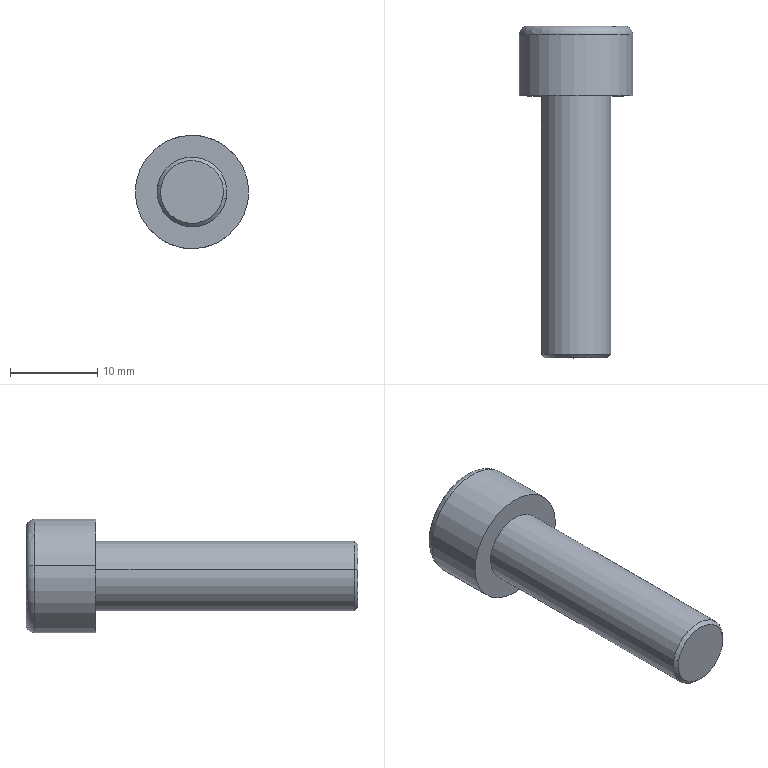Component | SolidWorks | hexagon socket head cap screws gb-25 | 1 solid | 25 faces | box 13 x 38 x 13 mm | volume 2418 mm3 | plane 15 | cone 4 | cylinder 4 | torus 2 | commonest cylinder face diameters 8 x2 13 x2
STEP:
#1=CARTESIAN_POINT('',(-5.304,20.394,23.936));
#2=VERTEX_POINT('',#1);
#3=CARTESIAN_POINT('',(-5.026,20.394,23.884));
#4=VERTEX_POINT('',#3);
#5=CARTESIAN_POINT('',(-5.165,20.394,23.91));
#6=DIRECTION('',(0.,-1.,0.));
#7=DIRECTION('',(-0.9828,0.,0.1847));
#8=AXIS2_PLACEMENT_3D('',#5,#6,#7);
#9=CIRCLE('',#8,0.1417);
#10=EDGE_CURVE('',#2,#4,#9,.T.);
#11=ORIENTED_EDGE('',*,*,#10,.F.);
#12=CARTESIAN_POINT('',(-5.32,20.41,23.939));
#13=VERTEX_POINT('',#12);
#14=CARTESIAN_POINT('',(-5.304,20.394,23.936));
#15=DIRECTION('',(-0.6949,0.7071,0.1306));
#16=VECTOR('',#15,39.37);
#17=LINE('',#14,#16);
#18=EDGE_CURVE('',#2,#13,#17,.T.);
#19=ORIENTED_EDGE('',*,*,#18,.T.);
#20=CARTESIAN_POINT('',(-5.01,20.41,23.881));
#21=VERTEX_POINT('',#20);
#22=CARTESIAN_POINT('',(-5.165,20.41,23.91));
#23=DIRECTION('',(0.,1.,0.));
#24=DIRECTION('',(-0.9828,0.,0.1847));
#25=AXIS2_PLACEMENT_3D('',#22,#23,#24);
#26=CIRCLE('',#25,0.1575);
#27=EDGE_CURVE('',#21,#13,#26,.T.);
#28=ORIENTED_EDGE('',*,*,#27,.F.);
#29=CARTESIAN_POINT('',(-5.026,20.394,23.884));
#30=DIRECTION('',(0.6949,0.7071,-0.1306));
#31=VECTOR('',#30,39.37);
#32=LINE('',#29,#31);
#33=EDGE_CURVE('',#4,#21,#32,.T.);
#34=ORIENTED_EDGE('',*,*,#33,.F.);
#35=EDGE_LOOP('',(#11,#19,#28,#34));
#36=FACE_OUTER_BOUND('',#35,.T.);
#37=CARTESIAN_POINT('',(-5.165,20.394,23.91));
#38=DIRECTION('',(0.,1.,0.));
#39=DIRECTION('',(0.9828,0.,-0.1847));
#40=AXIS2_PLACEMENT_3D('',#37,#38,#39);
#41=CONICAL_SURFACE('',#40,0.1417,0.7854);
#42=ADVANCED_FACE('',(#36),#41,.T.);
#43=CARTESIAN_POINT('',(-4.952,21.891,23.87));
#44=VERTEX_POINT('',#43);
#45=CARTESIAN_POINT('',(-5.378,21.891,23.95));
#46=VERTEX_POINT('',#45);
#47=CARTESIAN_POINT('',(-5.165,21.891,23.91));
#48=DIRECTION('',(0.,1.,0.));
#49=DIRECTION('',(-0.9828,0.,0.1847));
#50=AXIS2_PLACEMENT_3D('',#47,#48,#49);
#51=CIRCLE('',#50,0.2165);
#52=EDGE_CURVE('',#44,#46,#51,.T.);
#53=ORIENTED_EDGE('',*,*,#52,.F.);
#54=CARTESIAN_POINT('',(-4.913,21.851,23.863));
#55=VERTEX_POINT('',#54);
#56=CARTESIAN_POINT('',(-4.952,21.851,23.87));
#57=DIRECTION('',(-0.1847,0.,-0.9828));
#58=DIRECTION('',(-0.9828,0.,0.1847));
#59=AXIS2_PLACEMENT_3D('',#56,#57,#58);
#60=CIRCLE('',#59,0.03937);
#61=EDGE_CURVE('',#44,#55,#60,.T.);
#62=ORIENTED_EDGE('',*,*,#61,.T.);
#63=CARTESIAN_POINT('',(-5.416,21.851,23.957));
#64=VERTEX_POINT('',#63);
#65=CARTESIAN_POINT('',(-5.165,21.851,23.91));
#66=DIRECTION('',(0.,-1.,0.));
#67=DIRECTION('',(-0.9828,0.,0.1847));
#68=AXIS2_PLACEMENT_3D('',#65,#66,#67);
#69=CIRCLE('',#68,0.2559);
#70=EDGE_CURVE('',#64,#55,#69,.T.);
#71=ORIENTED_EDGE('',*,*,#70,.F.);
#72=CARTESIAN_POINT('',(-5.378,21.851,23.95));
#73=DIRECTION('',(0.1847,0.,0.9828));
#74=DIRECTION('',(0.9828,0.,-0.1847));
#75=AXIS2_PLACEMENT_3D('',#72,#73,#74);
#76=CIRCLE('',#75,0.03937);
#77=EDGE_CURVE('',#46,#64,#76,.T.);
#78=ORIENTED_EDGE('',*,*,#77,.F.);
#79=EDGE_LOOP('',(#53,#62,#71,#78));
#80=FACE_OUTER_BOUND('',#79,.T.);
#81=CARTESIAN_POINT('',(-5.165,21.851,23.91));
#82=DIRECTION('',(0.,-1.,0.));
#83=DIRECTION('',(-0.9828,0.,0.1847));
#84=AXIS2_PLACEMENT_3D('',#81,#82,#83);
#85=TOROIDAL_SURFACE('',#84,0.2165,0.03937);
#86=ADVANCED_FACE('',(#80),#85,.T.);
#87=CARTESIAN_POINT('',(-5.165,21.665,23.91));
#88=VERTEX_POINT('',#87);
#89=CARTESIAN_POINT('',(-5.049,21.733,23.888));
#90=VERTEX_POINT('',#89);
#91=CARTESIAN_POINT('',(-5.049,21.733,23.888));
#92=DIRECTION('',(0.8511,0.5,-0.16));
#93=VECTOR('',#92,39.37);
#94=LINE('',#91,#93);
#95=EDGE_CURVE('',#88,#90,#94,.T.);
#96=ORIENTED_EDGE('',*,*,#95,.F.);
#97=CARTESIAN_POINT('',(-5.281,21.733,23.932));
#98=VERTEX_POINT('',#97);
#99=CARTESIAN_POINT('',(-5.281,21.733,23.932));
#100=DIRECTION('',(-0.8511,0.5,0.16));
#101=VECTOR('',#100,39.37);
#102=LINE('',#99,#101);
#103=EDGE_CURVE('',#88,#98,#102,.T.);
#104=ORIENTED_EDGE('',*,*,#103,.T.);
#105=CARTESIAN_POINT('',(-5.255,21.733,23.987));
#106=VERTEX_POINT('',#105);
#107=CARTESIAN_POINT('',(-5.165,21.733,23.91));
#108=DIRECTION('',(0.,-1.,0.));
#109=DIRECTION('',(0.9828,0.,-0.1847));
#110=AXIS2_PLACEMENT_3D('',#107,#108,#109);
#111=CIRCLE('',#110,0.1181);
#112=EDGE_CURVE('',#106,#98,#111,.T.);
#113=ORIENTED_EDGE('',*,*,#112,.F.);
#114=CARTESIAN_POINT('',(-5.143,21.733,24.026));
#115=VERTEX_POINT('',#114);
#116=CARTESIAN_POINT('',(-5.165,21.733,23.91));
#117=DIRECTION('',(0.,-1.,0.));
#118=DIRECTION('',(0.9828,0.,-0.1847));
#119=AXIS2_PLACEMENT_3D('',#116,#117,#118);
#120=CIRCLE('',#119,0.1181);
#121=EDGE_CURVE('',#115,#106,#120,.T.);
#122=ORIENTED_EDGE('',*,*,#121,.F.);
#123=CARTESIAN_POINT('',(-5.054,21.733,23.949));
#124=VERTEX_POINT('',#123);
#125=CARTESIAN_POINT('',(-5.165,21.733,23.91));
#126=DIRECTION('',(0.,-1.,0.));
#127=DIRECTION('',(0.9828,0.,-0.1847));
#128=AXIS2_PLACEMENT_3D('',#125,#126,#127);
#129=CIRCLE('',#128,0.1181);
#130=EDGE_CURVE('',#124,#115,#129,.T.);
#131=ORIENTED_EDGE('',*,*,#130,.F.);
#132=CARTESIAN_POINT('',(-5.165,21.733,23.91));
#133=DIRECTION('',(0.,-1.,0.));
#134=DIRECTION('',(0.9828,0.,-0.1847));
#135=AXIS2_PLACEMENT_3D('',#132,#133,#134);
#136=CIRCLE('',#135,0.1181);
#137=EDGE_CURVE('',#90,#124,#136,.T.);
#138=ORIENTED_EDGE('',*,*,#137,.F.);
#139=EDGE_LOOP('',(#96,#104,#113,#122,#131,#138));
#140=FACE_OUTER_BOUND('',#139,.T.);
#141=CARTESIAN_POINT('',(-5.165,21.733,23.91));
#142=DIRECTION('',(0.,1.,0.));
#143=DIRECTION('',(0.9828,0.,-0.1847));
#144=AXIS2_PLACEMENT_3D('',#141,#142,#143);
#145=CONICAL_SURFACE('',#144,0.1181,1.047);
#146=ADVANCED_FACE('',(#140),#145,.F.);
#147=ORIENTED_EDGE('',*,*,#27,.T.);
#148=CARTESIAN_POINT('',(-5.32,21.576,23.939));
#149=VERTEX_POINT('',#148);
#150=CARTESIAN_POINT('',(-5.32,20.394,23.939));
#151=DIRECTION('',(0.,1.,0.));
#152=VECTOR('',#151,39.37);
#153=LINE('',#150,#152);
#154=EDGE_CURVE('',#13,#149,#153,.T.);
#155=ORIENTED_EDGE('',*,*,#154,.T.);
#156=CARTESIAN_POINT('',(-5.01,21.576,23.881));
#157=VERTEX_POINT('',#156);
#158=CARTESIAN_POINT('',(-5.165,21.576,23.91));
#159=DIRECTION('',(0.,-1.,0.));
#160=DIRECTION('',(-0.9828,0.,0.1847));
#161=AXIS2_PLACEMENT_3D('',#158,#159,#160);
#162=CIRCLE('',#161,0.1575);
#163=EDGE_CURVE('',#149,#157,#162,.T.);
#164=ORIENTED_EDGE('',*,*,#163,.T.);
#165=CARTESIAN_POINT('',(-5.01,20.394,23.881));
#166=DIRECTION('',(0.,1.,0.));
#167=VECTOR('',#166,39.37);
#168=LINE('',#165,#167);
#169=EDGE_CURVE('',#21,#157,#168,.T.);
#170=ORIENTED_EDGE('',*,*,#169,.F.);
#171=EDGE_LOOP('',(#147,#155,#164,#170));
#172=FACE_OUTER_BOUND('',#171,.T.);
#173=CARTESIAN_POINT('',(-5.165,20.394,23.91));
#174=DIRECTION('',(0.,1.,0.));
#175=DIRECTION('',(0.9828,0.,-0.1847));
#176=AXIS2_PLACEMENT_3D('',#173,#174,#175);
#177=CYLINDRICAL_SURFACE('',#176,0.1575);
#178=ADVANCED_FACE('',(#172),#177,.T.);
#179=CARTESIAN_POINT('',(-5.416,21.576,23.957));
#180=VERTEX_POINT('',#179);
#181=CARTESIAN_POINT('',(-4.913,21.576,23.863));
#182=VERTEX_POINT('',#181);
#183=CARTESIAN_POINT('',(-5.165,21.576,23.91));
#184=DIRECTION('',(0.,-1.,0.));
#185=DIRECTION('',(-0.9828,0.,0.1847));
#186=AXIS2_PLACEMENT_3D('',#183,#184,#185);
#187=CIRCLE('',#186,0.2559);
#188=EDGE_CURVE('',#180,#182,#187,.T.);
#189=ORIENTED_EDGE('',*,*,#188,.F.);
#190=CARTESIAN_POINT('',(-5.416,21.576,23.957));
#191=DIRECTION('',(0.,1.,0.));
#192=VECTOR('',#191,39.37);
#193=LINE('',#190,#192);
#194=EDGE_CURVE('',#180,#64,#193,.T.);
#195=ORIENTED_EDGE('',*,*,#194,.T.);
#196=ORIENTED_EDGE('',*,*,#70,.T.);
#197=CARTESIAN_POINT('',(-4.913,21.576,23.863));
#198=DIRECTION('',(0.,1.,0.));
#199=VECTOR('',#198,39.37);
#200=LINE('',#197,#199);
#201=EDGE_CURVE('',#182,#55,#200,.T.);
#202=ORIENTED_EDGE('',*,*,#201,.F.);
#203=EDGE_LOOP('',(#189,#195,#196,#202));
#204=FACE_OUTER_BOUND('',#203,.T.);
#205=CARTESIAN_POINT('',(-5.165,21.576,23.91));
#206=DIRECTION('',(0.,1.,0.));
#207=DIRECTION('',(0.9828,0.,-0.1847));
#208=AXIS2_PLACEMENT_3D('',#205,#206,#207);
#209=CYLINDRICAL_SURFACE('',#208,0.2559);
#210=ADVANCED_FACE('',(#204),#209,.T.);
#211=CARTESIAN_POINT('',(-5.076,21.733,24.013));
#212=VERTEX_POINT('',#211);
#213=CARTESIAN_POINT('',(-5.031,21.733,23.885));
#214=DIRECTION('',(-0.3314,0.,0.9435));
#215=VECTOR('',#214,39.37);
#216=LINE('',#213,#215);
#217=EDGE_CURVE('',#124,#212,#216,.T.);
#218=ORIENTED_EDGE('',*,*,#217,.F.);
#219=ORIENTED_EDGE('',*,*,#130,.T.);
#220=CARTESIAN_POINT('',(-5.076,21.733,24.013));
#221=DIRECTION('',(-0.9828,0.,0.1847));
#222=VECTOR('',#221,39.37);
#223=LINE('',#220,#222);
#224=EDGE_CURVE('',#212,#115,#223,.T.);
#225=ORIENTED_EDGE('',*,*,#224,.F.);
#226=EDGE_LOOP('',(#218,#219,#225));
#227=FACE_OUTER_BOUND('',#226,.T.);
#228=CARTESIAN_POINT('',(-5.121,21.733,24.142));
#229=DIRECTION('',(0.,1.,0.));
#230=DIRECTION('',(0.9828,0.,-0.1847));
#231=AXIS2_PLACEMENT_3D('',#228,#229,#230);
#232=PLANE('',#231);
#233=ADVANCED_FACE('',(#227),#232,.T.);
#234=CARTESIAN_POINT('',(-5.21,21.733,24.039));
#235=VERTEX_POINT('',#234);
#236=CARTESIAN_POINT('',(-5.076,21.733,24.013));
#237=DIRECTION('',(-0.9828,0.,0.1847));
#238=VECTOR('',#237,39.37);
#239=LINE('',#236,#238);
#240=EDGE_CURVE('',#115,#235,#239,.T.);
#241=ORIENTED_EDGE('',*,*,#240,.F.);
#242=ORIENTED_EDGE('',*,*,#121,.T.);
#243=CARTESIAN_POINT('',(-5.21,21.733,24.039));
#244=DIRECTION('',(-0.6513,0.,-0.7588));
#245=VECTOR('',#244,39.37);
#246=LINE('',#243,#245);
#247=EDGE_CURVE('',#235,#106,#246,.T.);
#248=ORIENTED_EDGE('',*,*,#247,.F.);
#249=EDGE_LOOP('',(#241,#242,#248));
#250=FACE_OUTER_BOUND('',#249,.T.);
#251=CARTESIAN_POINT('',(-5.121,21.733,24.142));
#252=DIRECTION('',(0.,1.,0.));
#253=DIRECTION('',(0.9828,0.,-0.1847));
#254=AXIS2_PLACEMENT_3D('',#251,#252,#253);
#255=PLANE('',#254);
#256=ADVANCED_FACE('',(#250),#255,.T.);
#257=CARTESIAN_POINT('',(-5.299,21.733,23.935));
#258=VERTEX_POINT('',#257);
#259=CARTESIAN_POINT('',(-5.21,21.733,24.039));
#260=DIRECTION('',(-0.6513,0.,-0.7588));
#261=VECTOR('',#260,39.37);
#262=LINE('',#259,#261);
#263=EDGE_CURVE('',#106,#258,#262,.T.);
#264=ORIENTED_EDGE('',*,*,#263,.F.);
#265=ORIENTED_EDGE('',*,*,#112,.T.);
#266=CARTESIAN_POINT('',(-5.276,21.733,23.871));
#267=VERTEX_POINT('',#266);
#268=CARTESIAN_POINT('',(-5.165,21.733,23.91));
#269=DIRECTION('',(0.,-1.,0.));
#270=DIRECTION('',(0.9828,0.,-0.1847));
#271=AXIS2_PLACEMENT_3D('',#268,#269,#270);
#272=CIRCLE('',#271,0.1181);
#273=EDGE_CURVE('',#98,#267,#272,.T.);
#274=ORIENTED_EDGE('',*,*,#273,.T.);
#275=CARTESIAN_POINT('',(-5.299,21.733,23.935));
#276=DIRECTION('',(0.3314,0.,-0.9435));
#277=VECTOR('',#276,39.37);
#278=LINE('',#275,#277);
#279=EDGE_CURVE('',#258,#267,#278,.T.);
#280=ORIENTED_EDGE('',*,*,#279,.F.);
#281=EDGE_LOOP('',(#264,#265,#274,#280));
#282=FACE_OUTER_BOUND('',#281,.T.);
#283=CARTESIAN_POINT('',(-5.121,21.733,24.142));
#284=DIRECTION('',(0.,1.,0.));
#285=DIRECTION('',(0.9828,0.,-0.1847));
#286=AXIS2_PLACEMENT_3D('',#283,#284,#285);
#287=PLANE('',#286);
#288=ADVANCED_FACE('',(#282),#287,.T.);
#289=CARTESIAN_POINT('',(-5.254,21.733,23.806));
#290=VERTEX_POINT('',#289);
#291=CARTESIAN_POINT('',(-5.299,21.733,23.935));
#292=DIRECTION('',(0.3314,0.,-0.9435));
#293=VECTOR('',#292,39.37);
#294=LINE('',#291,#293);
#295=EDGE_CURVE('',#267,#290,#294,.T.);
#296=ORIENTED_EDGE('',*,*,#295,.F.);
#297=CARTESIAN_POINT('',(-5.187,21.733,23.794));
#298=VERTEX_POINT('',#297);
#299=CARTESIAN_POINT('',(-5.165,21.733,23.91));
#300=DIRECTION('',(0.,-1.,0.));
#301=DIRECTION('',(-0.9828,0.,0.1847));
#302=AXIS2_PLACEMENT_3D('',#299,#300,#301);
#303=CIRCLE('',#302,0.1181);
#304=EDGE_CURVE('',#267,#298,#303,.T.);
#305=ORIENTED_EDGE('',*,*,#304,.T.);
#306=CARTESIAN_POINT('',(-5.254,21.733,23.806));
#307=DIRECTION('',(0.9828,0.,-0.1847));
#308=VECTOR('',#307,39.37);
#309=LINE('',#306,#308);
#310=EDGE_CURVE('',#290,#298,#309,.T.);
#311=ORIENTED_EDGE('',*,*,#310,.F.);
#312=EDGE_LOOP('',(#296,#305,#311));
#313=FACE_OUTER_BOUND('',#312,.T.);
#314=CARTESIAN_POINT('',(-5.121,21.733,24.142));
#315=DIRECTION('',(0.,1.,0.));
#316=DIRECTION('',(0.9828,0.,-0.1847));
#317=AXIS2_PLACEMENT_3D('',#314,#315,#316);
#318=PLANE('',#317);
#319=ADVANCED_FACE('',(#313),#318,.T.);
#320=CARTESIAN_POINT('',(-5.12,21.733,23.781));
#321=VERTEX_POINT('',#320);
#322=CARTESIAN_POINT('',(-5.254,21.733,23.806));
#323=DIRECTION('',(0.9828,0.,-0.1847));
#324=VECTOR('',#323,39.37);
#325=LINE('',#322,#324);
#326=EDGE_CURVE('',#298,#321,#325,.T.);
#327=ORIENTED_EDGE('',*,*,#326,.F.);
#328=CARTESIAN_POINT('',(-5.075,21.733,23.833));
#329=VERTEX_POINT('',#328);
#330=CARTESIAN_POINT('',(-5.165,21.733,23.91));
#331=DIRECTION('',(0.,-1.,0.));
#332=DIRECTION('',(0.9828,0.,-0.1847));
#333=AXIS2_PLACEMENT_3D('',#330,#331,#332);
#334=CIRCLE('',#333,0.1181);
#335=EDGE_CURVE('',#298,#329,#334,.T.);
#336=ORIENTED_EDGE('',*,*,#335,.T.);
#337=CARTESIAN_POINT('',(-5.12,21.733,23.781));
#338=DIRECTION('',(0.6513,0.,0.7588));
#339=VECTOR('',#338,39.37);
#340=LINE('',#337,#339);
#341=EDGE_CURVE('',#321,#329,#340,.T.);
#342=ORIENTED_EDGE('',*,*,#341,.F.);
#343=EDGE_LOOP('',(#327,#336,#342));
#344=FACE_OUTER_BOUND('',#343,.T.);
#345=CARTESIAN_POINT('',(-5.121,21.733,24.142));
#346=DIRECTION('',(0.,1.,0.));
#347=DIRECTION('',(0.9828,0.,-0.1847));
#348=AXIS2_PLACEMENT_3D('',#345,#346,#347);
#349=PLANE('',#348);
#350=ADVANCED_FACE('',(#344),#349,.T.);
#351=CARTESIAN_POINT('',(-5.031,21.733,23.885));
#352=VERTEX_POINT('',#351);
#353=CARTESIAN_POINT('',(-5.12,21.733,23.781));
#354=DIRECTION('',(0.6513,0.,0.7588));
#355=VECTOR('',#354,39.37);
#356=LINE('',#353,#355);
#357=EDGE_CURVE('',#329,#352,#356,.T.);
#358=ORIENTED_EDGE('',*,*,#357,.F.);
#359=CARTESIAN_POINT('',(-5.165,21.733,23.91));
#360=DIRECTION('',(0.,-1.,0.));
#361=DIRECTION('',(0.9828,0.,-0.1847));
#362=AXIS2_PLACEMENT_3D('',#359,#360,#361);
#363=CIRCLE('',#362,0.1181);
#364=EDGE_CURVE('',#329,#90,#363,.T.);
#365=ORIENTED_EDGE('',*,*,#364,.T.);
#366=ORIENTED_EDGE('',*,*,#137,.T.);
#367=CARTESIAN_POINT('',(-5.031,21.733,23.885));
#368=DIRECTION('',(-0.3314,0.,0.9435));
#369=VECTOR('',#368,39.37);
#370=LINE('',#367,#369);
#371=EDGE_CURVE('',#352,#124,#370,.T.);
#372=ORIENTED_EDGE('',*,*,#371,.F.);
#373=EDGE_LOOP('',(#358,#365,#366,#372));
#374=FACE_OUTER_BOUND('',#373,.T.);
#375=CARTESIAN_POINT('',(-5.121,21.733,24.142));
#376=DIRECTION('',(0.,1.,0.));
#377=DIRECTION('',(0.9828,0.,-0.1847));
#378=AXIS2_PLACEMENT_3D('',#375,#376,#377);
#379=PLANE('',#378);
#380=ADVANCED_FACE('',(#374),#379,.T.);
#381=CARTESIAN_POINT('',(-5.165,21.891,23.91));
#382=DIRECTION('',(0.,1.,0.));
#383=DIRECTION('',(-0.9828,0.,0.1847));
#384=AXIS2_PLACEMENT_3D('',#381,#382,#383);
#385=CIRCLE('',#384,0.2165);
#386=EDGE_CURVE('',#46,#44,#385,.T.);
#387=ORIENTED_EDGE('',*,*,#386,.T.);
#388=ORIENTED_EDGE('',*,*,#52,.T.);
#389=EDGE_LOOP('',(#387,#388));
#390=FACE_OUTER_BOUND('',#389,.T.);
#391=CARTESIAN_POINT('',(-5.21,21.891,24.039));
#392=VERTEX_POINT('',#391);
#393=CARTESIAN_POINT('',(-5.299,21.891,23.935));
#394=VERTEX_POINT('',#393);
#395=CARTESIAN_POINT('',(-5.21,21.891,24.039));
#396=DIRECTION('',(-0.6513,0.,-0.7588));
#397=VECTOR('',#396,39.37);
#398=LINE('',#395,#397);
#399=EDGE_CURVE('',#392,#394,#398,.T.);
#400=ORIENTED_EDGE('',*,*,#399,.T.);
#401=CARTESIAN_POINT('',(-5.254,21.891,23.806));
#402=VERTEX_POINT('',#401);
#403=CARTESIAN_POINT('',(-5.299,21.891,23.935));
#404=DIRECTION('',(0.3314,0.,-0.9435));
#405=VECTOR('',#404,39.37);
#406=LINE('',#403,#405);
#407=EDGE_CURVE('',#394,#402,#406,.T.);
#408=ORIENTED_EDGE('',*,*,#407,.T.);
#409=CARTESIAN_POINT('',(-5.12,21.891,23.781));
#410=VERTEX_POINT('',#409);
#411=CARTESIAN_POINT('',(-5.254,21.891,23.806));
#412=DIRECTION('',(0.9828,0.,-0.1847));
#413=VECTOR('',#412,39.37);
#414=LINE('',#411,#413);
#415=EDGE_CURVE('',#402,#410,#414,.T.);
#416=ORIENTED_EDGE('',*,*,#415,.T.);
#417=CARTESIAN_POINT('',(-5.031,21.891,23.885));
#418=VERTEX_POINT('',#417);
#419=CARTESIAN_POINT('',(-5.12,21.891,23.781));
#420=DIRECTION('',(0.6513,0.,0.7588));
#421=VECTOR('',#420,39.37);
#422=LINE('',#419,#421);
#423=EDGE_CURVE('',#410,#418,#422,.T.);
#424=ORIENTED_EDGE('',*,*,#423,.T.);
#425=CARTESIAN_POINT('',(-5.076,21.891,24.013));
#426=VERTEX_POINT('',#425);
#427=CARTESIAN_POINT('',(-5.031,21.891,23.885));
#428=DIRECTION('',(-0.3314,0.,0.9435));
#429=VECTOR('',#428,39.37);
#430=LINE('',#427,#429);
#431=EDGE_CURVE('',#418,#426,#430,.T.);
#432=ORIENTED_EDGE('',*,*,#431,.T.);
#433=CARTESIAN_POINT('',(-5.076,21.891,24.013));
#434=DIRECTION('',(-0.9828,0.,0.1847));
#435=VECTOR('',#434,39.37);
#436=LINE('',#433,#435);
#437=EDGE_CURVE('',#426,#392,#436,.T.);
#438=ORIENTED_EDGE('',*,*,#437,.T.);
#439=EDGE_LOOP('',(#400,#408,#416,#424,#432,#438));
#440=FACE_BOUND('',#439,.T.);
#441=CARTESIAN_POINT('',(-5.165,21.891,23.91));
#442=DIRECTION('',(0.,-1.,0.));
#443=DIRECTION('',(-0.9828,0.,0.1847));
#444=AXIS2_PLACEMENT_3D('',#441,#442,#443);
#445=PLANE('',#444);
#446=ADVANCED_FACE('',(#390,#440),#445,.F.);
#447=CARTESIAN_POINT('',(-5.165,21.576,23.91));
#448=DIRECTION('',(0.,-1.,0.));
#449=DIRECTION('',(-0.9828,0.,0.1847));
#450=AXIS2_PLACEMENT_3D('',#447,#448,#449);
#451=CIRCLE('',#450,0.2559);
#452=EDGE_CURVE('',#182,#180,#451,.T.);
#453=ORIENTED_EDGE('',*,*,#452,.T.);
#454=ORIENTED_EDGE('',*,*,#188,.T.);
#455=EDGE_LOOP('',(#453,#454));
#456=FACE_OUTER_BOUND('',#455,.T.);
#457=CARTESIAN_POINT('',(-5.165,21.576,23.91));
#458=DIRECTION('',(0.,-1.,0.));
#459=DIRECTION('',(-0.9828,0.,0.1847));
#460=AXIS2_PLACEMENT_3D('',#457,#458,#459);
#461=CIRCLE('',#460,0.1575);
#462=EDGE_CURVE('',#157,#149,#461,.T.);
#463=ORIENTED_EDGE('',*,*,#462,.F.);
#464=ORIENTED_EDGE('',*,*,#163,.F.);
#465=EDGE_LOOP('',(#463,#464));
#466=FACE_BOUND('',#465,.T.);
#467=CARTESIAN_POINT('',(-5.165,21.576,23.91));
#468=DIRECTION('',(0.,-1.,0.));
#469=DIRECTION('',(-0.9828,0.,0.1847));
#470=AXIS2_PLACEMENT_3D('',#467,#468,#469);
#471=PLANE('',#470);
#472=ADVANCED_FACE('',(#456,#466),#471,.T.);
#473=ORIENTED_EDGE('',*,*,#194,.F.);
#474=ORIENTED_EDGE('',*,*,#452,.F.);
#475=ORIENTED_EDGE('',*,*,#201,.T.);
#476=CARTESIAN_POINT('',(-5.165,21.851,23.91));
#477=DIRECTION('',(0.,-1.,0.));
#478=DIRECTION('',(-0.9828,0.,0.1847));
#479=AXIS2_PLACEMENT_3D('',#476,#477,#478);
#480=CIRCLE('',#479,0.2559);
#481=EDGE_CURVE('',#55,#64,#480,.T.);
#482=ORIENTED_EDGE('',*,*,#481,.T.);
#483=EDGE_LOOP('',(#473,#474,#475,#482));
#484=FACE_OUTER_BOUND('',#483,.T.);
#485=CARTESIAN_POINT('',(-5.165,21.576,23.91));
#486=DIRECTION('',(0.,1.,0.));
#487=DIRECTION('',(0.9828,0.,-0.1847));
#488=AXIS2_PLACEMENT_3D('',#485,#486,#487);
#489=CYLINDRICAL_SURFACE('',#488,0.2559);
#490=ADVANCED_FACE('',(#484),#489,.T.);
#491=ORIENTED_EDGE('',*,*,#154,.F.);
#492=CARTESIAN_POINT('',(-5.165,20.41,23.91));
#493=DIRECTION('',(0.,1.,0.));
#494=DIRECTION('',(-0.9828,0.,0.1847));
#495=AXIS2_PLACEMENT_3D('',#492,#493,#494);
#496=CIRCLE('',#495,0.1575);
#497=EDGE_CURVE('',#13,#21,#496,.T.);
#498=ORIENTED_EDGE('',*,*,#497,.T.);
#499=ORIENTED_EDGE('',*,*,#169,.T.);
#500=ORIENTED_EDGE('',*,*,#462,.T.);
#501=EDGE_LOOP('',(#491,#498,#499,#500));
#502=FACE_OUTER_BOUND('',#501,.T.);
#503=CARTESIAN_POINT('',(-5.165,20.394,23.91));
#504=DIRECTION('',(0.,1.,0.));
#505=DIRECTION('',(0.9828,0.,-0.1847));
#506=AXIS2_PLACEMENT_3D('',#503,#504,#505);
#507=CYLINDRICAL_SURFACE('',#506,0.1575);
#508=ADVANCED_FACE('',(#502),#507,.T.);
#509=CARTESIAN_POINT('',(-5.165,20.394,23.91));
#510=DIRECTION('',(0.,-1.,0.));
#511=DIRECTION('',(-0.9828,0.,0.1847));
#512=AXIS2_PLACEMENT_3D('',#509,#510,#511);
#513=CIRCLE('',#512,0.1417);
#514=EDGE_CURVE('',#4,#2,#513,.T.);
#515=ORIENTED_EDGE('',*,*,#514,.T.);
#516=ORIENTED_EDGE('',*,*,#10,.T.);
#517=EDGE_LOOP('',(#515,#516));
#518=FACE_OUTER_BOUND('',#517,.T.);
#519=CARTESIAN_POINT('',(-5.165,20.394,23.91));
#520=DIRECTION('',(0.,-1.,0.));
#521=DIRECTION('',(-0.9828,0.,0.1847));
#522=AXIS2_PLACEMENT_3D('',#519,#520,#521);
#523=PLANE('',#522);
#524=ADVANCED_FACE('',(#518),#523,.T.);
#525=ORIENTED_EDGE('',*,*,#399,.F.);
#526=CARTESIAN_POINT('',(-5.21,21.733,24.039));
#527=DIRECTION('',(0.,1.,0.));
#528=VECTOR('',#527,39.37);
#529=LINE('',#526,#528);
#530=EDGE_CURVE('',#235,#392,#529,.T.);
#531=ORIENTED_EDGE('',*,*,#530,.F.);
#532=ORIENTED_EDGE('',*,*,#247,.T.);
#533=ORIENTED_EDGE('',*,*,#263,.T.);
#534=CARTESIAN_POINT('',(-5.299,21.733,23.935));
#535=DIRECTION('',(0.,1.,0.));
#536=VECTOR('',#535,39.37);
#537=LINE('',#534,#536);
#538=EDGE_CURVE('',#258,#394,#537,.T.);
#539=ORIENTED_EDGE('',*,*,#538,.T.);
#540=EDGE_LOOP('',(#525,#531,#532,#533,#539));
#541=FACE_OUTER_BOUND('',#540,.T.);
#542=CARTESIAN_POINT('',(-5.21,21.733,24.039));
#543=DIRECTION('',(0.7588,0.,-0.6513));
#544=DIRECTION('',(0.6513,0.,0.7588));
#545=AXIS2_PLACEMENT_3D('',#542,#543,#544);
#546=PLANE('',#545);
#547=ADVANCED_FACE('',(#541),#546,.T.);
#548=ORIENTED_EDGE('',*,*,#407,.F.);
#549=ORIENTED_EDGE('',*,*,#538,.F.);
#550=ORIENTED_EDGE('',*,*,#279,.T.);
#551=ORIENTED_EDGE('',*,*,#295,.T.);
#552=CARTESIAN_POINT('',(-5.254,21.733,23.806));
#553=DIRECTION('',(0.,1.,0.));
#554=VECTOR('',#553,39.37);
#555=LINE('',#552,#554);
#556=EDGE_CURVE('',#290,#402,#555,.T.);
#557=ORIENTED_EDGE('',*,*,#556,.T.);
#558=EDGE_LOOP('',(#548,#549,#550,#551,#557));
#559=FACE_OUTER_BOUND('',#558,.T.);
#560=CARTESIAN_POINT('',(-5.299,21.733,23.935));
#561=DIRECTION('',(0.9435,0.,0.3314));
#562=DIRECTION('',(-0.3314,0.,0.9435));
#563=AXIS2_PLACEMENT_3D('',#560,#561,#562);
#564=PLANE('',#563);
#565=ADVANCED_FACE('',(#559),#564,.T.);
#566=ORIENTED_EDGE('',*,*,#415,.F.);
#567=ORIENTED_EDGE('',*,*,#556,.F.);
#568=ORIENTED_EDGE('',*,*,#310,.T.);
#569=ORIENTED_EDGE('',*,*,#326,.T.);
#570=CARTESIAN_POINT('',(-5.12,21.733,23.781));
#571=DIRECTION('',(0.,1.,0.));
#572=VECTOR('',#571,39.37);
#573=LINE('',#570,#572);
#574=EDGE_CURVE('',#321,#410,#573,.T.);
#575=ORIENTED_EDGE('',*,*,#574,.T.);
#576=EDGE_LOOP('',(#566,#567,#568,#569,#575));
#577=FACE_OUTER_BOUND('',#576,.T.);
#578=CARTESIAN_POINT('',(-5.254,21.733,23.806));
#579=DIRECTION('',(0.1847,0.,0.9828));
#580=DIRECTION('',(-0.9828,0.,0.1847));
#581=AXIS2_PLACEMENT_3D('',#578,#579,#580);
#582=PLANE('',#581);
#583=ADVANCED_FACE('',(#577),#582,.T.);
#584=ORIENTED_EDGE('',*,*,#423,.F.);
#585=ORIENTED_EDGE('',*,*,#574,.F.);
#586=ORIENTED_EDGE('',*,*,#341,.T.);
#587=ORIENTED_EDGE('',*,*,#357,.T.);
#588=CARTESIAN_POINT('',(-5.031,21.733,23.885));
#589=DIRECTION('',(0.,1.,0.));
#590=VECTOR('',#589,39.37);
#591=LINE('',#588,#590);
#592=EDGE_CURVE('',#352,#418,#591,.T.);
#593=ORIENTED_EDGE('',*,*,#592,.T.);
#594=EDGE_LOOP('',(#584,#585,#586,#587,#593));
#595=FACE_OUTER_BOUND('',#594,.T.);
#596=CARTESIAN_POINT('',(-5.12,21.733,23.781));
#597=DIRECTION('',(-0.7588,0.,0.6513));
#598=DIRECTION('',(-0.6513,0.,-0.7588));
#599=AXIS2_PLACEMENT_3D('',#596,#597,#598);
#600=PLANE('',#599);
#601=ADVANCED_FACE('',(#595),#600,.T.);
#602=ORIENTED_EDGE('',*,*,#431,.F.);
#603=ORIENTED_EDGE('',*,*,#592,.F.);
#604=ORIENTED_EDGE('',*,*,#371,.T.);
#605=ORIENTED_EDGE('',*,*,#217,.T.);
#606=CARTESIAN_POINT('',(-5.076,21.733,24.013));
#607=DIRECTION('',(0.,1.,0.));
#608=VECTOR('',#607,39.37);
#609=LINE('',#606,#608);
#610=EDGE_CURVE('',#212,#426,#609,.T.);
#611=ORIENTED_EDGE('',*,*,#610,.T.);
#612=EDGE_LOOP('',(#602,#603,#604,#605,#611));
#613=FACE_OUTER_BOUND('',#612,.T.);
#614=CARTESIAN_POINT('',(-5.031,21.733,23.885));
#615=DIRECTION('',(-0.9435,0.,-0.3314));
#616=DIRECTION('',(0.3314,0.,-0.9435));
#617=AXIS2_PLACEMENT_3D('',#614,#615,#616);
#618=PLANE('',#617);
#619=ADVANCED_FACE('',(#613),#618,.T.);
#620=ORIENTED_EDGE('',*,*,#437,.F.);
#621=ORIENTED_EDGE('',*,*,#610,.F.);
#622=ORIENTED_EDGE('',*,*,#224,.T.);
#623=ORIENTED_EDGE('',*,*,#240,.T.);
#624=ORIENTED_EDGE('',*,*,#530,.T.);
#625=EDGE_LOOP('',(#620,#621,#622,#623,#624));
#626=FACE_OUTER_BOUND('',#625,.T.);
#627=CARTESIAN_POINT('',(-5.076,21.733,24.013));
#628=DIRECTION('',(-0.1847,0.,-0.9828));
#629=DIRECTION('',(0.9828,0.,-0.1847));
#630=AXIS2_PLACEMENT_3D('',#627,#628,#629);
#631=PLANE('',#630);
#632=ADVANCED_FACE('',(#626),#631,.T.);
#633=ORIENTED_EDGE('',*,*,#103,.F.);
#634=ORIENTED_EDGE('',*,*,#95,.T.);
#635=ORIENTED_EDGE('',*,*,#364,.F.);
#636=ORIENTED_EDGE('',*,*,#335,.F.);
#637=ORIENTED_EDGE('',*,*,#304,.F.);
#638=ORIENTED_EDGE('',*,*,#273,.F.);
#639=EDGE_LOOP('',(#633,#634,#635,#636,#637,#638));
#640=FACE_OUTER_BOUND('',#639,.T.);
#641=CARTESIAN_POINT('',(-5.165,21.733,23.91));
#642=DIRECTION('',(0.,1.,0.));
#643=DIRECTION('',(0.9828,0.,-0.1847));
#644=AXIS2_PLACEMENT_3D('',#641,#642,#643);
#645=CONICAL_SURFACE('',#644,0.1181,1.047);
#646=ADVANCED_FACE('',(#640),#645,.F.);
#647=ORIENTED_EDGE('',*,*,#61,.F.);
#648=ORIENTED_EDGE('',*,*,#386,.F.);
#649=ORIENTED_EDGE('',*,*,#77,.T.);
#650=ORIENTED_EDGE('',*,*,#481,.F.);
#651=EDGE_LOOP('',(#647,#648,#649,#650));
#652=FACE_OUTER_BOUND('',#651,.T.);
#653=CARTESIAN_POINT('',(-5.165,21.851,23.91));
#654=DIRECTION('',(0.,-1.,0.));
#655=DIRECTION('',(-0.9828,0.,0.1847));
#656=AXIS2_PLACEMENT_3D('',#653,#654,#655);
#657=TOROIDAL_SURFACE('',#656,0.2165,0.03937);
#658=ADVANCED_FACE('',(#652),#657,.T.);
#659=ORIENTED_EDGE('',*,*,#18,.F.);
#660=ORIENTED_EDGE('',*,*,#514,.F.);
#661=ORIENTED_EDGE('',*,*,#33,.T.);
#662=ORIENTED_EDGE('',*,*,#497,.F.);
#663=EDGE_LOOP('',(#659,#660,#661,#662));
#664=FACE_OUTER_BOUND('',#663,.T.);
#665=CARTESIAN_POINT('',(-5.165,20.394,23.91));
#666=DIRECTION('',(0.,1.,0.));
#667=DIRECTION('',(0.9828,0.,-0.1847));
#668=AXIS2_PLACEMENT_3D('',#665,#666,#667);
#669=CONICAL_SURFACE('',#668,0.1417,0.7854);
#670=ADVANCED_FACE('',(#664),#669,.T.);
#671=CLOSED_SHELL('',(#42,#86,#146,#178,#210,#233,#256,#288,#319,#350,#380,#446,#472,#490,#508,#524,#547,#565,#583,#601,#619,#632,#646,#658,#670));
#672=MANIFOLD_SOLID_BREP('',#671);
#673=CARTESIAN_POINT('',(0.,0.,0.));
#674=DIRECTION('',(0.,0.,1.));
#675=DIRECTION('',(1.,0.,0.));
#676=AXIS2_PLACEMENT_3D('',#673,#674,#675);
#677=(LENGTH_UNIT()NAMED_UNIT(*)SI_UNIT($,.METRE.));
#678=LENGTH_MEASURE_WITH_UNIT(LENGTH_MEASURE(0.0254),#677);
#679=DIMENSIONAL_EXPONENTS(1.,0.,0.,0.,0.,0.,0.);
#680=(CONVERSION_BASED_UNIT('',#678)LENGTH_UNIT()NAMED_UNIT(#679));
#681=UNCERTAINTY_MEASURE_WITH_UNIT(LENGTH_MEASURE(0.00001),#680,'','');
#682=(NAMED_UNIT(*)PLANE_ANGLE_UNIT()SI_UNIT($,.RADIAN.));
#683=(NAMED_UNIT(*)SI_UNIT($,.STERADIAN.)SOLID_ANGLE_UNIT());
#684=(GEOMETRIC_REPRESENTATION_CONTEXT(3)GLOBAL_UNCERTAINTY_ASSIGNED_CONTEXT((#681))GLOBAL_UNIT_ASSIGNED_CONTEXT((#680,#682,#683))REPRESENTATION_CONTEXT('',''));
#685=ADVANCED_BREP_SHAPE_REPRESENTATION('',(#672,#676),#684);
#686=COLOUR_RGB('',0.7922,0.8196,0.9333);
#687=FILL_AREA_STYLE_COLOUR('',#686);
#688=FILL_AREA_STYLE('',(#687));
#689=SURFACE_STYLE_FILL_AREA(#688);
#690=SURFACE_SIDE_STYLE('',(#689));
#691=SURFACE_STYLE_USAGE(.BOTH.,#690);
#692=PRESENTATION_STYLE_ASSIGNMENT((#691));
#693=STYLED_ITEM('',(#692),#672);
#694=(LENGTH_UNIT()NAMED_UNIT(*)SI_UNIT($,.METRE.));
#695=LENGTH_MEASURE_WITH_UNIT(LENGTH_MEASURE(0.0254),#694);
#696=DIMENSIONAL_EXPONENTS(1.,0.,0.,0.,0.,0.,0.);
#697=(CONVERSION_BASED_UNIT('',#695)LENGTH_UNIT()NAMED_UNIT(#696));
#698=UNCERTAINTY_MEASURE_WITH_UNIT(LENGTH_MEASURE(0.00001),#697,'','');
#699=(NAMED_UNIT(*)PLANE_ANGLE_UNIT()SI_UNIT($,.RADIAN.));
#700=(NAMED_UNIT(*)SI_UNIT($,.STERADIAN.)SOLID_ANGLE_UNIT());
#701=(GEOMETRIC_REPRESENTATION_CONTEXT(3)GLOBAL_UNCERTAINTY_ASSIGNED_CONTEXT((#698))GLOBAL_UNIT_ASSIGNED_CONTEXT((#697,#699,#700))REPRESENTATION_CONTEXT('',''));
#702=MECHANICAL_DESIGN_GEOMETRIC_PRESENTATION_REPRESENTATION('',(#693),#701);
#703=PRESENTATION_LAYER_ASSIGNMENT('','',(#693));